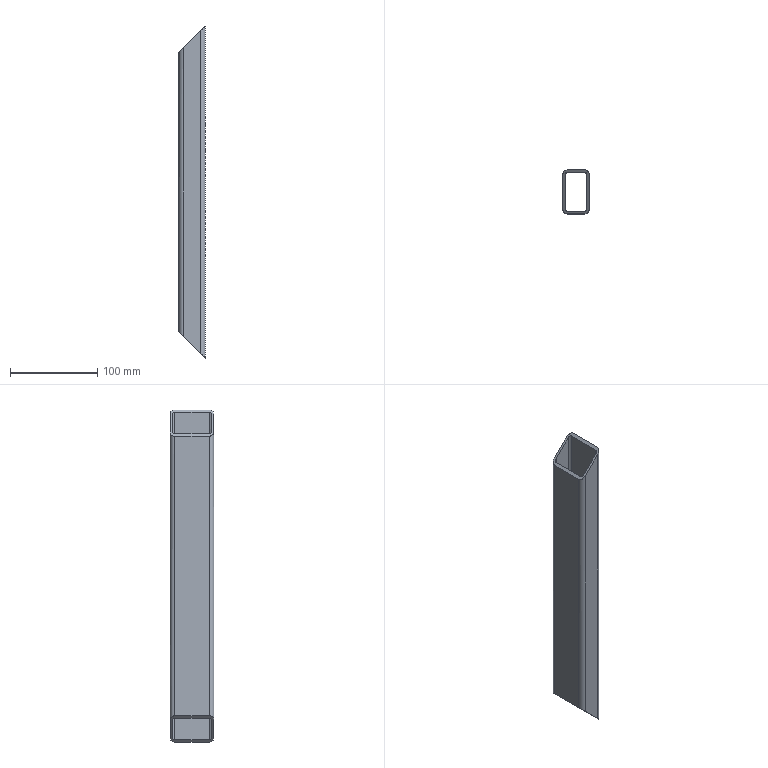Component | SolidWorks | Frame-1_SquareTube2-1 | 1 solid | 18 faces | box 30 x 50 x 380 mm | volume 130043 mm3 | plane 10 | cylinder 8 | commonest cylinder face diameters 10.4 x4 5.2 x4
STEP:
#1=COLOUR_RGB('',0.7922,0.8196,0.9333);
#2=FILL_AREA_STYLE_COLOUR('',#1);
#3=FILL_AREA_STYLE('',(#2));
#4=SURFACE_STYLE_FILL_AREA(#3);
#5=SURFACE_SIDE_STYLE('',(#4));
#6=SURFACE_STYLE_USAGE(.BOTH.,#5);
#7=PRESENTATION_STYLE_ASSIGNMENT((#6));
#8=CARTESIAN_POINT('',(20.276,-0.7795,-7.48));
#9=VERTEX_POINT('',#8);
#10=CARTESIAN_POINT('',(20.276,-0.7795,7.48));
#11=VERTEX_POINT('',#10);
#12=CARTESIAN_POINT('',(20.276,-0.7795,-6.89));
#13=DIRECTION('',(0.,0.,1.));
#14=VECTOR('',#13,39.37);
#15=LINE('',#12,#14);
#16=EDGE_CURVE('',#9,#11,#15,.T.);
#17=ORIENTED_EDGE('',*,*,#16,.F.);
#18=CARTESIAN_POINT('',(20.276,0.7795,-7.48));
#19=VERTEX_POINT('',#18);
#20=CARTESIAN_POINT('',(20.276,-0.7795,-7.48));
#21=DIRECTION('',(0.,-1.,0.));
#22=VECTOR('',#21,39.37);
#23=LINE('',#20,#22);
#24=EDGE_CURVE('',#19,#9,#23,.T.);
#25=ORIENTED_EDGE('',*,*,#24,.F.);
#26=CARTESIAN_POINT('',(20.276,0.7795,7.48));
#27=VERTEX_POINT('',#26);
#28=CARTESIAN_POINT('',(20.276,0.7795,-6.89));
#29=DIRECTION('',(0.,0.,-1.));
#30=VECTOR('',#29,39.37);
#31=LINE('',#28,#30);
#32=EDGE_CURVE('',#27,#19,#31,.T.);
#33=ORIENTED_EDGE('',*,*,#32,.F.);
#34=CARTESIAN_POINT('',(20.276,-0.7795,7.48));
#35=DIRECTION('',(0.,1.,0.));
#36=VECTOR('',#35,39.37);
#37=LINE('',#34,#36);
#38=EDGE_CURVE('',#11,#27,#37,.T.);
#39=ORIENTED_EDGE('',*,*,#38,.F.);
#40=EDGE_LOOP('',(#17,#25,#33,#39));
#41=FACE_OUTER_BOUND('',#40,.T.);
#42=CARTESIAN_POINT('',(20.276,-0.7795,-6.89));
#43=DIRECTION('',(-1.,0.,0.));
#44=DIRECTION('',(0.,0.,1.));
#45=AXIS2_PLACEMENT_3D('',#42,#43,#44);
#46=PLANE('',#45);
#47=ADVANCED_FACE('',(#41),#46,.F.);
#48=ORIENTED_EDGE('',*,*,#38,.T.);
#49=CARTESIAN_POINT('',(20.071,0.9843,7.276));
#50=VERTEX_POINT('',#49);
#51=CARTESIAN_POINT('',(20.276,0.7795,7.48));
#52=CARTESIAN_POINT('',(20.276,0.8995,7.48));
#53=CARTESIAN_POINT('',(20.191,0.9843,7.396));
#54=CARTESIAN_POINT('',(20.071,0.9843,7.276));
#55=(BOUNDED_CURVE()B_SPLINE_CURVE(3,(#51,#52,#53,#54),.UNSPECIFIED.,.F.,.F.)B_SPLINE_CURVE_WITH_KNOTS((4,4),(0.,1.571),.UNSPECIFIED.)CURVE()GEOMETRIC_REPRESENTATION_ITEM()RATIONAL_B_SPLINE_CURVE((1.,0.8047,0.8047,1.))REPRESENTATION_ITEM(''));
#56=EDGE_CURVE('',#27,#50,#55,.T.);
#57=ORIENTED_EDGE('',*,*,#56,.T.);
#58=CARTESIAN_POINT('',(19.299,0.9843,6.504));
#59=VERTEX_POINT('',#58);
#60=CARTESIAN_POINT('',(19.685,0.9843,6.89));
#61=DIRECTION('',(-0.7071,0.,-0.7071));
#62=VECTOR('',#61,39.37);
#63=LINE('',#60,#62);
#64=EDGE_CURVE('',#50,#59,#63,.T.);
#65=ORIENTED_EDGE('',*,*,#64,.T.);
#66=CARTESIAN_POINT('',(19.094,0.7795,6.299));
#67=VERTEX_POINT('',#66);
#68=CARTESIAN_POINT('',(19.299,0.9843,6.504));
#69=CARTESIAN_POINT('',(19.179,0.9843,6.384));
#70=CARTESIAN_POINT('',(19.094,0.8995,6.299));
#71=CARTESIAN_POINT('',(19.094,0.7795,6.299));
#72=(BOUNDED_CURVE()B_SPLINE_CURVE(3,(#68,#69,#70,#71),.UNSPECIFIED.,.F.,.T.)B_SPLINE_CURVE_WITH_KNOTS((4,4),(1.571,3.142),.UNSPECIFIED.)CURVE()GEOMETRIC_REPRESENTATION_ITEM()RATIONAL_B_SPLINE_CURVE((1.,0.8047,0.8047,1.))REPRESENTATION_ITEM(''));
#73=EDGE_CURVE('',#59,#67,#72,.T.);
#74=ORIENTED_EDGE('',*,*,#73,.T.);
#75=CARTESIAN_POINT('',(19.094,-0.7795,6.299));
#76=VERTEX_POINT('',#75);
#77=CARTESIAN_POINT('',(19.094,0.,6.299));
#78=DIRECTION('',(0.,-1.,0.));
#79=VECTOR('',#78,39.37);
#80=LINE('',#77,#79);
#81=EDGE_CURVE('',#67,#76,#80,.T.);
#82=ORIENTED_EDGE('',*,*,#81,.T.);
#83=CARTESIAN_POINT('',(19.299,-0.9843,6.504));
#84=VERTEX_POINT('',#83);
#85=CARTESIAN_POINT('',(19.094,-0.7795,6.299));
#86=CARTESIAN_POINT('',(19.094,-0.8995,6.299));
#87=CARTESIAN_POINT('',(19.179,-0.9843,6.384));
#88=CARTESIAN_POINT('',(19.299,-0.9843,6.504));
#89=(BOUNDED_CURVE()B_SPLINE_CURVE(3,(#85,#86,#87,#88),.UNSPECIFIED.,.F.,.F.)B_SPLINE_CURVE_WITH_KNOTS((4,4),(3.142,4.712),.UNSPECIFIED.)CURVE()GEOMETRIC_REPRESENTATION_ITEM()RATIONAL_B_SPLINE_CURVE((1.,0.8047,0.8047,1.))REPRESENTATION_ITEM(''));
#90=EDGE_CURVE('',#76,#84,#89,.T.);
#91=ORIENTED_EDGE('',*,*,#90,.T.);
#92=CARTESIAN_POINT('',(20.071,-0.9843,7.276));
#93=VERTEX_POINT('',#92);
#94=CARTESIAN_POINT('',(19.685,-0.9843,6.89));
#95=DIRECTION('',(0.7071,0.,0.7071));
#96=VECTOR('',#95,39.37);
#97=LINE('',#94,#96);
#98=EDGE_CURVE('',#84,#93,#97,.T.);
#99=ORIENTED_EDGE('',*,*,#98,.T.);
#100=CARTESIAN_POINT('',(20.071,-0.9843,7.276));
#101=CARTESIAN_POINT('',(20.191,-0.9843,7.396));
#102=CARTESIAN_POINT('',(20.276,-0.8995,7.48));
#103=CARTESIAN_POINT('',(20.276,-0.7795,7.48));
#104=(BOUNDED_CURVE()B_SPLINE_CURVE(3,(#100,#101,#102,#103),.UNSPECIFIED.,.F.,.F.)B_SPLINE_CURVE_WITH_KNOTS((4,4),(4.712,6.283),.UNSPECIFIED.)CURVE()GEOMETRIC_REPRESENTATION_ITEM()RATIONAL_B_SPLINE_CURVE((1.,0.8047,0.8047,1.))REPRESENTATION_ITEM(''));
#105=EDGE_CURVE('',#93,#11,#104,.T.);
#106=ORIENTED_EDGE('',*,*,#105,.T.);
#107=EDGE_LOOP('',(#48,#57,#65,#74,#82,#91,#99,#106));
#108=FACE_OUTER_BOUND('',#107,.T.);
#109=CARTESIAN_POINT('',(19.197,0.7795,6.402));
#110=VERTEX_POINT('',#109);
#111=CARTESIAN_POINT('',(19.299,0.8819,6.504));
#112=VERTEX_POINT('',#111);
#113=CARTESIAN_POINT('',(19.197,0.7795,6.402));
#114=CARTESIAN_POINT('',(19.197,0.8395,6.402));
#115=CARTESIAN_POINT('',(19.239,0.8819,6.444));
#116=CARTESIAN_POINT('',(19.299,0.8819,6.504));
#117=(BOUNDED_CURVE()B_SPLINE_CURVE(3,(#113,#114,#115,#116),.UNSPECIFIED.,.F.,.F.)B_SPLINE_CURVE_WITH_KNOTS((4,4),(3.142,4.712),.UNSPECIFIED.)CURVE()GEOMETRIC_REPRESENTATION_ITEM()RATIONAL_B_SPLINE_CURVE((1.,0.8047,0.8047,1.))REPRESENTATION_ITEM(''));
#118=EDGE_CURVE('',#110,#112,#117,.T.);
#119=ORIENTED_EDGE('',*,*,#118,.T.);
#120=CARTESIAN_POINT('',(20.071,0.8819,7.276));
#121=VERTEX_POINT('',#120);
#122=CARTESIAN_POINT('',(19.685,0.8819,6.89));
#123=DIRECTION('',(0.7071,0.,0.7071));
#124=VECTOR('',#123,39.37);
#125=LINE('',#122,#124);
#126=EDGE_CURVE('',#112,#121,#125,.T.);
#127=ORIENTED_EDGE('',*,*,#126,.T.);
#128=CARTESIAN_POINT('',(20.173,0.7795,7.378));
#129=VERTEX_POINT('',#128);
#130=CARTESIAN_POINT('',(20.071,0.8819,7.276));
#131=CARTESIAN_POINT('',(20.131,0.8819,7.336));
#132=CARTESIAN_POINT('',(20.173,0.8395,7.378));
#133=CARTESIAN_POINT('',(20.173,0.7795,7.378));
#134=(BOUNDED_CURVE()B_SPLINE_CURVE(3,(#130,#131,#132,#133),.UNSPECIFIED.,.F.,.F.)B_SPLINE_CURVE_WITH_KNOTS((4,4),(4.712,6.283),.UNSPECIFIED.)CURVE()GEOMETRIC_REPRESENTATION_ITEM()RATIONAL_B_SPLINE_CURVE((1.,0.8047,0.8047,1.))REPRESENTATION_ITEM(''));
#135=EDGE_CURVE('',#121,#129,#134,.T.);
#136=ORIENTED_EDGE('',*,*,#135,.T.);
#137=CARTESIAN_POINT('',(20.173,-0.7795,7.378));
#138=VERTEX_POINT('',#137);
#139=CARTESIAN_POINT('',(20.173,0.,7.378));
#140=DIRECTION('',(0.,-1.,0.));
#141=VECTOR('',#140,39.37);
#142=LINE('',#139,#141);
#143=EDGE_CURVE('',#129,#138,#142,.T.);
#144=ORIENTED_EDGE('',*,*,#143,.T.);
#145=CARTESIAN_POINT('',(20.071,-0.8819,7.276));
#146=VERTEX_POINT('',#145);
#147=CARTESIAN_POINT('',(20.173,-0.7795,7.378));
#148=CARTESIAN_POINT('',(20.173,-0.8395,7.378));
#149=CARTESIAN_POINT('',(20.131,-0.8819,7.336));
#150=CARTESIAN_POINT('',(20.071,-0.8819,7.276));
#151=(BOUNDED_CURVE()B_SPLINE_CURVE(3,(#147,#148,#149,#150),.UNSPECIFIED.,.F.,.F.)B_SPLINE_CURVE_WITH_KNOTS((4,4),(0.,1.571),.UNSPECIFIED.)CURVE()GEOMETRIC_REPRESENTATION_ITEM()RATIONAL_B_SPLINE_CURVE((1.,0.8047,0.8047,1.))REPRESENTATION_ITEM(''));
#152=EDGE_CURVE('',#138,#146,#151,.T.);
#153=ORIENTED_EDGE('',*,*,#152,.T.);
#154=CARTESIAN_POINT('',(19.299,-0.8819,6.504));
#155=VERTEX_POINT('',#154);
#156=CARTESIAN_POINT('',(19.685,-0.8819,6.89));
#157=DIRECTION('',(-0.7071,0.,-0.7071));
#158=VECTOR('',#157,39.37);
#159=LINE('',#156,#158);
#160=EDGE_CURVE('',#146,#155,#159,.T.);
#161=ORIENTED_EDGE('',*,*,#160,.T.);
#162=CARTESIAN_POINT('',(19.197,-0.7795,6.402));
#163=VERTEX_POINT('',#162);
#164=CARTESIAN_POINT('',(19.299,-0.8819,6.504));
#165=CARTESIAN_POINT('',(19.239,-0.8819,6.444));
#166=CARTESIAN_POINT('',(19.197,-0.8395,6.402));
#167=CARTESIAN_POINT('',(19.197,-0.7795,6.402));
#168=(BOUNDED_CURVE()B_SPLINE_CURVE(3,(#164,#165,#166,#167),.UNSPECIFIED.,.F.,.F.)B_SPLINE_CURVE_WITH_KNOTS((4,4),(1.571,3.142),.UNSPECIFIED.)CURVE()GEOMETRIC_REPRESENTATION_ITEM()RATIONAL_B_SPLINE_CURVE((1.,0.8047,0.8047,1.))REPRESENTATION_ITEM(''));
#169=EDGE_CURVE('',#155,#163,#168,.T.);
#170=ORIENTED_EDGE('',*,*,#169,.T.);
#171=CARTESIAN_POINT('',(19.197,0.,6.402));
#172=DIRECTION('',(0.,1.,0.));
#173=VECTOR('',#172,39.37);
#174=LINE('',#171,#173);
#175=EDGE_CURVE('',#163,#110,#174,.T.);
#176=ORIENTED_EDGE('',*,*,#175,.T.);
#177=EDGE_LOOP('',(#119,#127,#136,#144,#153,#161,#170,#176));
#178=FACE_BOUND('',#177,.T.);
#179=CARTESIAN_POINT('',(19.685,0.,6.89));
#180=DIRECTION('',(-0.7071,0.,0.7071));
#181=DIRECTION('',(0.7071,0.,0.7071));
#182=AXIS2_PLACEMENT_3D('',#179,#180,#181);
#183=PLANE('',#182);
#184=ADVANCED_FACE('',(#108,#178),#183,.T.);
#185=CARTESIAN_POINT('',(20.071,-0.9843,-7.276));
#186=VERTEX_POINT('',#185);
#187=CARTESIAN_POINT('',(20.071,-0.9843,-7.276));
#188=CARTESIAN_POINT('',(20.191,-0.9843,-7.396));
#189=CARTESIAN_POINT('',(20.276,-0.8995,-7.48));
#190=CARTESIAN_POINT('',(20.276,-0.7795,-7.48));
#191=(BOUNDED_CURVE()B_SPLINE_CURVE(3,(#187,#188,#189,#190),.UNSPECIFIED.,.F.,.F.)B_SPLINE_CURVE_WITH_KNOTS((4,4),(1.571,3.142),.UNSPECIFIED.)CURVE()GEOMETRIC_REPRESENTATION_ITEM()RATIONAL_B_SPLINE_CURVE((1.,0.8047,0.8047,1.))REPRESENTATION_ITEM(''));
#192=EDGE_CURVE('',#186,#9,#191,.T.);
#193=ORIENTED_EDGE('',*,*,#192,.T.);
#194=ORIENTED_EDGE('',*,*,#16,.T.);
#195=ORIENTED_EDGE('',*,*,#105,.F.);
#196=CARTESIAN_POINT('',(20.071,-0.9843,-6.89));
#197=DIRECTION('',(0.,0.,-1.));
#198=VECTOR('',#197,39.37);
#199=LINE('',#196,#198);
#200=EDGE_CURVE('',#93,#186,#199,.T.);
#201=ORIENTED_EDGE('',*,*,#200,.T.);
#202=EDGE_LOOP('',(#193,#194,#195,#201));
#203=FACE_OUTER_BOUND('',#202,.T.);
#204=CARTESIAN_POINT('',(20.071,-0.7795,-6.89));
#205=DIRECTION('',(0.,0.,1.));
#206=DIRECTION('',(1.,0.,0.));
#207=AXIS2_PLACEMENT_3D('',#204,#205,#206);
#208=CYLINDRICAL_SURFACE('',#207,0.2047);
#209=ADVANCED_FACE('',(#203),#208,.T.);
#210=CARTESIAN_POINT('',(19.299,-0.9843,-6.504));
#211=VERTEX_POINT('',#210);
#212=CARTESIAN_POINT('',(19.685,-0.9843,-6.89));
#213=DIRECTION('',(-0.7071,0.,0.7071));
#214=VECTOR('',#213,39.37);
#215=LINE('',#212,#214);
#216=EDGE_CURVE('',#186,#211,#215,.T.);
#217=ORIENTED_EDGE('',*,*,#216,.T.);
#218=CARTESIAN_POINT('',(19.094,-0.7795,-6.299));
#219=VERTEX_POINT('',#218);
#220=CARTESIAN_POINT('',(19.299,-0.9843,-6.504));
#221=CARTESIAN_POINT('',(19.179,-0.9843,-6.384));
#222=CARTESIAN_POINT('',(19.094,-0.8995,-6.299));
#223=CARTESIAN_POINT('',(19.094,-0.7795,-6.299));
#224=(BOUNDED_CURVE()B_SPLINE_CURVE(3,(#220,#221,#222,#223),.UNSPECIFIED.,.F.,.F.)B_SPLINE_CURVE_WITH_KNOTS((4,4),(4.712,6.283),.UNSPECIFIED.)CURVE()GEOMETRIC_REPRESENTATION_ITEM()RATIONAL_B_SPLINE_CURVE((1.,0.8047,0.8047,1.))REPRESENTATION_ITEM(''));
#225=EDGE_CURVE('',#211,#219,#224,.T.);
#226=ORIENTED_EDGE('',*,*,#225,.T.);
#227=CARTESIAN_POINT('',(19.094,0.7795,-6.299));
#228=VERTEX_POINT('',#227);
#229=CARTESIAN_POINT('',(19.094,0.,-6.299));
#230=DIRECTION('',(0.,1.,0.));
#231=VECTOR('',#230,39.37);
#232=LINE('',#229,#231);
#233=EDGE_CURVE('',#219,#228,#232,.T.);
#234=ORIENTED_EDGE('',*,*,#233,.T.);
#235=CARTESIAN_POINT('',(19.299,0.9843,-6.504));
#236=VERTEX_POINT('',#235);
#237=CARTESIAN_POINT('',(19.094,0.7795,-6.299));
#238=CARTESIAN_POINT('',(19.094,0.8995,-6.299));
#239=CARTESIAN_POINT('',(19.179,0.9843,-6.384));
#240=CARTESIAN_POINT('',(19.299,0.9843,-6.504));
#241=(BOUNDED_CURVE()B_SPLINE_CURVE(3,(#237,#238,#239,#240),.UNSPECIFIED.,.F.,.F.)B_SPLINE_CURVE_WITH_KNOTS((4,4),(0.,1.571),.UNSPECIFIED.)CURVE()GEOMETRIC_REPRESENTATION_ITEM()RATIONAL_B_SPLINE_CURVE((1.,0.8047,0.8047,1.))REPRESENTATION_ITEM(''));
#242=EDGE_CURVE('',#228,#236,#241,.T.);
#243=ORIENTED_EDGE('',*,*,#242,.T.);
#244=CARTESIAN_POINT('',(20.071,0.9843,-7.276));
#245=VERTEX_POINT('',#244);
#246=CARTESIAN_POINT('',(19.685,0.9843,-6.89));
#247=DIRECTION('',(0.7071,0.,-0.7071));
#248=VECTOR('',#247,39.37);
#249=LINE('',#246,#248);
#250=EDGE_CURVE('',#236,#245,#249,.T.);
#251=ORIENTED_EDGE('',*,*,#250,.T.);
#252=CARTESIAN_POINT('',(20.071,0.9843,-7.276));
#253=CARTESIAN_POINT('',(20.191,0.9843,-7.396));
#254=CARTESIAN_POINT('',(20.276,0.8995,-7.48));
#255=CARTESIAN_POINT('',(20.276,0.7795,-7.48));
#256=(BOUNDED_CURVE()B_SPLINE_CURVE(3,(#252,#253,#254,#255),.UNSPECIFIED.,.F.,.T.)B_SPLINE_CURVE_WITH_KNOTS((4,4),(1.571,3.142),.UNSPECIFIED.)CURVE()GEOMETRIC_REPRESENTATION_ITEM()RATIONAL_B_SPLINE_CURVE((1.,0.8047,0.8047,1.))REPRESENTATION_ITEM(''));
#257=EDGE_CURVE('',#245,#19,#256,.T.);
#258=ORIENTED_EDGE('',*,*,#257,.T.);
#259=ORIENTED_EDGE('',*,*,#24,.T.);
#260=ORIENTED_EDGE('',*,*,#192,.F.);
#261=EDGE_LOOP('',(#217,#226,#234,#243,#251,#258,#259,#260));
#262=FACE_OUTER_BOUND('',#261,.T.);
#263=CARTESIAN_POINT('',(20.071,-0.8819,-7.276));
#264=VERTEX_POINT('',#263);
#265=CARTESIAN_POINT('',(20.173,-0.7795,-7.378));
#266=VERTEX_POINT('',#265);
#267=CARTESIAN_POINT('',(20.071,-0.8819,-7.276));
#268=CARTESIAN_POINT('',(20.131,-0.8819,-7.336));
#269=CARTESIAN_POINT('',(20.173,-0.8395,-7.378));
#270=CARTESIAN_POINT('',(20.173,-0.7795,-7.378));
#271=(BOUNDED_CURVE()B_SPLINE_CURVE(3,(#267,#268,#269,#270),.UNSPECIFIED.,.F.,.F.)B_SPLINE_CURVE_WITH_KNOTS((4,4),(1.571,3.142),.UNSPECIFIED.)CURVE()GEOMETRIC_REPRESENTATION_ITEM()RATIONAL_B_SPLINE_CURVE((1.,0.8047,0.8047,1.))REPRESENTATION_ITEM(''));
#272=EDGE_CURVE('',#264,#266,#271,.T.);
#273=ORIENTED_EDGE('',*,*,#272,.T.);
#274=CARTESIAN_POINT('',(20.173,0.7795,-7.378));
#275=VERTEX_POINT('',#274);
#276=CARTESIAN_POINT('',(20.173,0.,-7.378));
#277=DIRECTION('',(0.,1.,0.));
#278=VECTOR('',#277,39.37);
#279=LINE('',#276,#278);
#280=EDGE_CURVE('',#266,#275,#279,.T.);
#281=ORIENTED_EDGE('',*,*,#280,.T.);
#282=CARTESIAN_POINT('',(20.071,0.8819,-7.276));
#283=VERTEX_POINT('',#282);
#284=CARTESIAN_POINT('',(20.173,0.7795,-7.378));
#285=CARTESIAN_POINT('',(20.173,0.8395,-7.378));
#286=CARTESIAN_POINT('',(20.131,0.8819,-7.336));
#287=CARTESIAN_POINT('',(20.071,0.8819,-7.276));
#288=(BOUNDED_CURVE()B_SPLINE_CURVE(3,(#284,#285,#286,#287),.UNSPECIFIED.,.F.,.F.)B_SPLINE_CURVE_WITH_KNOTS((4,4),(3.142,4.712),.UNSPECIFIED.)CURVE()GEOMETRIC_REPRESENTATION_ITEM()RATIONAL_B_SPLINE_CURVE((1.,0.8047,0.8047,1.))REPRESENTATION_ITEM(''));
#289=EDGE_CURVE('',#275,#283,#288,.T.);
#290=ORIENTED_EDGE('',*,*,#289,.T.);
#291=CARTESIAN_POINT('',(19.299,0.8819,-6.504));
#292=VERTEX_POINT('',#291);
#293=CARTESIAN_POINT('',(19.685,0.8819,-6.89));
#294=DIRECTION('',(-0.7071,0.,0.7071));
#295=VECTOR('',#294,39.37);
#296=LINE('',#293,#295);
#297=EDGE_CURVE('',#283,#292,#296,.T.);
#298=ORIENTED_EDGE('',*,*,#297,.T.);
#299=CARTESIAN_POINT('',(19.197,0.7795,-6.402));
#300=VERTEX_POINT('',#299);
#301=CARTESIAN_POINT('',(19.299,0.8819,-6.504));
#302=CARTESIAN_POINT('',(19.239,0.8819,-6.444));
#303=CARTESIAN_POINT('',(19.197,0.8395,-6.402));
#304=CARTESIAN_POINT('',(19.197,0.7795,-6.402));
#305=(BOUNDED_CURVE()B_SPLINE_CURVE(3,(#301,#302,#303,#304),.UNSPECIFIED.,.F.,.F.)B_SPLINE_CURVE_WITH_KNOTS((4,4),(4.712,6.283),.UNSPECIFIED.)CURVE()GEOMETRIC_REPRESENTATION_ITEM()RATIONAL_B_SPLINE_CURVE((1.,0.8047,0.8047,1.))REPRESENTATION_ITEM(''));
#306=EDGE_CURVE('',#292,#300,#305,.T.);
#307=ORIENTED_EDGE('',*,*,#306,.T.);
#308=CARTESIAN_POINT('',(19.197,-0.7795,-6.402));
#309=VERTEX_POINT('',#308);
#310=CARTESIAN_POINT('',(19.197,0.,-6.402));
#311=DIRECTION('',(0.,-1.,0.));
#312=VECTOR('',#311,39.37);
#313=LINE('',#310,#312);
#314=EDGE_CURVE('',#300,#309,#313,.T.);
#315=ORIENTED_EDGE('',*,*,#314,.T.);
#316=CARTESIAN_POINT('',(19.299,-0.8819,-6.504));
#317=VERTEX_POINT('',#316);
#318=CARTESIAN_POINT('',(19.197,-0.7795,-6.402));
#319=CARTESIAN_POINT('',(19.197,-0.8395,-6.402));
#320=CARTESIAN_POINT('',(19.239,-0.8819,-6.444));
#321=CARTESIAN_POINT('',(19.299,-0.8819,-6.504));
#322=(BOUNDED_CURVE()B_SPLINE_CURVE(3,(#318,#319,#320,#321),.UNSPECIFIED.,.F.,.F.)B_SPLINE_CURVE_WITH_KNOTS((4,4),(0.,1.571),.UNSPECIFIED.)CURVE()GEOMETRIC_REPRESENTATION_ITEM()RATIONAL_B_SPLINE_CURVE((1.,0.8047,0.8047,1.))REPRESENTATION_ITEM(''));
#323=EDGE_CURVE('',#309,#317,#322,.T.);
#324=ORIENTED_EDGE('',*,*,#323,.T.);
#325=CARTESIAN_POINT('',(19.685,-0.8819,-6.89));
#326=DIRECTION('',(0.7071,0.,-0.7071));
#327=VECTOR('',#326,39.37);
#328=LINE('',#325,#327);
#329=EDGE_CURVE('',#317,#264,#328,.T.);
#330=ORIENTED_EDGE('',*,*,#329,.T.);
#331=EDGE_LOOP('',(#273,#281,#290,#298,#307,#315,#324,#330));
#332=FACE_BOUND('',#331,.T.);
#333=CARTESIAN_POINT('',(19.685,0.,-6.89));
#334=DIRECTION('',(-0.7071,0.,-0.7071));
#335=DIRECTION('',(-0.7071,0.,0.7071));
#336=AXIS2_PLACEMENT_3D('',#333,#334,#335);
#337=PLANE('',#336);
#338=ADVANCED_FACE('',(#262,#332),#337,.T.);
#339=ORIENTED_EDGE('',*,*,#257,.F.);
#340=CARTESIAN_POINT('',(20.071,0.9843,-6.89));
#341=DIRECTION('',(0.,0.,1.));
#342=VECTOR('',#341,39.37);
#343=LINE('',#340,#342);
#344=EDGE_CURVE('',#245,#50,#343,.T.);
#345=ORIENTED_EDGE('',*,*,#344,.T.);
#346=ORIENTED_EDGE('',*,*,#56,.F.);
#347=ORIENTED_EDGE('',*,*,#32,.T.);
#348=EDGE_LOOP('',(#339,#345,#346,#347));
#349=FACE_OUTER_BOUND('',#348,.T.);
#350=CARTESIAN_POINT('',(20.071,0.7795,-6.89));
#351=DIRECTION('',(0.,0.,1.));
#352=DIRECTION('',(1.,0.,0.));
#353=AXIS2_PLACEMENT_3D('',#350,#351,#352);
#354=CYLINDRICAL_SURFACE('',#353,0.2047);
#355=ADVANCED_FACE('',(#349),#354,.T.);
#356=CARTESIAN_POINT('',(19.299,-0.9843,-6.89));
#357=DIRECTION('',(0.,0.,1.));
#358=VECTOR('',#357,39.37);
#359=LINE('',#356,#358);
#360=EDGE_CURVE('',#211,#84,#359,.T.);
#361=ORIENTED_EDGE('',*,*,#360,.F.);
#362=ORIENTED_EDGE('',*,*,#216,.F.);
#363=ORIENTED_EDGE('',*,*,#200,.F.);
#364=ORIENTED_EDGE('',*,*,#98,.F.);
#365=EDGE_LOOP('',(#361,#362,#363,#364));
#366=FACE_OUTER_BOUND('',#365,.T.);
#367=CARTESIAN_POINT('',(20.071,-0.9843,-6.89));
#368=DIRECTION('',(0.,1.,0.));
#369=DIRECTION('',(0.,0.,1.));
#370=AXIS2_PLACEMENT_3D('',#367,#368,#369);
#371=PLANE('',#370);
#372=ADVANCED_FACE('',(#366),#371,.F.);
#373=ORIENTED_EDGE('',*,*,#225,.F.);
#374=ORIENTED_EDGE('',*,*,#360,.T.);
#375=ORIENTED_EDGE('',*,*,#90,.F.);
#376=CARTESIAN_POINT('',(19.094,-0.7795,-6.89));
#377=DIRECTION('',(0.,0.,-1.));
#378=VECTOR('',#377,39.37);
#379=LINE('',#376,#378);
#380=EDGE_CURVE('',#76,#219,#379,.T.);
#381=ORIENTED_EDGE('',*,*,#380,.T.);
#382=EDGE_LOOP('',(#373,#374,#375,#381));
#383=FACE_OUTER_BOUND('',#382,.T.);
#384=CARTESIAN_POINT('',(19.299,-0.7795,-6.89));
#385=DIRECTION('',(0.,0.,1.));
#386=DIRECTION('',(1.,0.,0.));
#387=AXIS2_PLACEMENT_3D('',#384,#385,#386);
#388=CYLINDRICAL_SURFACE('',#387,0.2047);
#389=ADVANCED_FACE('',(#383),#388,.T.);
#390=CARTESIAN_POINT('',(19.094,0.7795,-6.89));
#391=DIRECTION('',(0.,0.,1.));
#392=VECTOR('',#391,39.37);
#393=LINE('',#390,#392);
#394=EDGE_CURVE('',#228,#67,#393,.T.);
#395=ORIENTED_EDGE('',*,*,#394,.F.);
#396=ORIENTED_EDGE('',*,*,#233,.F.);
#397=ORIENTED_EDGE('',*,*,#380,.F.);
#398=ORIENTED_EDGE('',*,*,#81,.F.);
#399=EDGE_LOOP('',(#395,#396,#397,#398));
#400=FACE_OUTER_BOUND('',#399,.T.);
#401=CARTESIAN_POINT('',(19.094,0.7795,-6.89));
#402=DIRECTION('',(1.,0.,0.));
#403=DIRECTION('',(0.,0.,-1.));
#404=AXIS2_PLACEMENT_3D('',#401,#402,#403);
#405=PLANE('',#404);
#406=ADVANCED_FACE('',(#400),#405,.F.);
#407=ORIENTED_EDGE('',*,*,#242,.F.);
#408=ORIENTED_EDGE('',*,*,#394,.T.);
#409=ORIENTED_EDGE('',*,*,#73,.F.);
#410=CARTESIAN_POINT('',(19.299,0.9843,-6.89));
#411=DIRECTION('',(0.,0.,-1.));
#412=VECTOR('',#411,39.37);
#413=LINE('',#410,#412);
#414=EDGE_CURVE('',#59,#236,#413,.T.);
#415=ORIENTED_EDGE('',*,*,#414,.T.);
#416=EDGE_LOOP('',(#407,#408,#409,#415));
#417=FACE_OUTER_BOUND('',#416,.T.);
#418=CARTESIAN_POINT('',(19.299,0.7795,-6.89));
#419=DIRECTION('',(0.,0.,1.));
#420=DIRECTION('',(1.,0.,0.));
#421=AXIS2_PLACEMENT_3D('',#418,#419,#420);
#422=CYLINDRICAL_SURFACE('',#421,0.2047);
#423=ADVANCED_FACE('',(#417),#422,.T.);
#424=ORIENTED_EDGE('',*,*,#344,.F.);
#425=ORIENTED_EDGE('',*,*,#250,.F.);
#426=ORIENTED_EDGE('',*,*,#414,.F.);
#427=ORIENTED_EDGE('',*,*,#64,.F.);
#428=EDGE_LOOP('',(#424,#425,#426,#427));
#429=FACE_OUTER_BOUND('',#428,.T.);
#430=CARTESIAN_POINT('',(19.299,0.9843,-6.89));
#431=DIRECTION('',(0.,-1.,0.));
#432=DIRECTION('',(0.,0.,-1.));
#433=AXIS2_PLACEMENT_3D('',#430,#431,#432);
#434=PLANE('',#433);
#435=ADVANCED_FACE('',(#429),#434,.F.);
#436=CARTESIAN_POINT('',(19.299,0.8819,-6.89));
#437=DIRECTION('',(0.,0.,-1.));
#438=VECTOR('',#437,39.37);
#439=LINE('',#436,#438);
#440=EDGE_CURVE('',#112,#292,#439,.T.);
#441=ORIENTED_EDGE('',*,*,#440,.T.);
#442=ORIENTED_EDGE('',*,*,#297,.F.);
#443=CARTESIAN_POINT('',(20.071,0.8819,-6.89));
#444=DIRECTION('',(0.,0.,1.));
#445=VECTOR('',#444,39.37);
#446=LINE('',#443,#445);
#447=EDGE_CURVE('',#283,#121,#446,.T.);
#448=ORIENTED_EDGE('',*,*,#447,.T.);
#449=ORIENTED_EDGE('',*,*,#126,.F.);
#450=EDGE_LOOP('',(#441,#442,#448,#449));
#451=FACE_OUTER_BOUND('',#450,.T.);
#452=CARTESIAN_POINT('',(19.299,0.8819,-6.89));
#453=DIRECTION('',(0.,-1.,0.));
#454=DIRECTION('',(0.,0.,-1.));
#455=AXIS2_PLACEMENT_3D('',#452,#453,#454);
#456=PLANE('',#455);
#457=ADVANCED_FACE('',(#451),#456,.T.);
#458=ORIENTED_EDGE('',*,*,#118,.F.);
#459=CARTESIAN_POINT('',(19.197,0.7795,-6.89));
#460=DIRECTION('',(0.,0.,1.));
#461=VECTOR('',#460,39.37);
#462=LINE('',#459,#461);
#463=EDGE_CURVE('',#300,#110,#462,.T.);
#464=ORIENTED_EDGE('',*,*,#463,.F.);
#465=ORIENTED_EDGE('',*,*,#306,.F.);
#466=ORIENTED_EDGE('',*,*,#440,.F.);
#467=EDGE_LOOP('',(#458,#464,#465,#466));
#468=FACE_OUTER_BOUND('',#467,.T.);
#469=CARTESIAN_POINT('',(19.299,0.7795,-6.89));
#470=DIRECTION('',(0.,0.,1.));
#471=DIRECTION('',(1.,0.,0.));
#472=AXIS2_PLACEMENT_3D('',#469,#470,#471);
#473=CYLINDRICAL_SURFACE('',#472,0.1024);
#474=ADVANCED_FACE('',(#468),#473,.F.);
#475=CARTESIAN_POINT('',(19.197,-0.7795,-6.89));
#476=DIRECTION('',(0.,0.,-1.));
#477=VECTOR('',#476,39.37);
#478=LINE('',#475,#477);
#479=EDGE_CURVE('',#163,#309,#478,.T.);
#480=ORIENTED_EDGE('',*,*,#479,.T.);
#481=ORIENTED_EDGE('',*,*,#314,.F.);
#482=ORIENTED_EDGE('',*,*,#463,.T.);
#483=ORIENTED_EDGE('',*,*,#175,.F.);
#484=EDGE_LOOP('',(#480,#481,#482,#483));
#485=FACE_OUTER_BOUND('',#484,.T.);
#486=CARTESIAN_POINT('',(19.197,0.7795,-6.89));
#487=DIRECTION('',(1.,0.,0.));
#488=DIRECTION('',(0.,0.,-1.));
#489=AXIS2_PLACEMENT_3D('',#486,#487,#488);
#490=PLANE('',#489);
#491=ADVANCED_FACE('',(#485),#490,.T.);
#492=ORIENTED_EDGE('',*,*,#169,.F.);
#493=CARTESIAN_POINT('',(19.299,-0.8819,-6.89));
#494=DIRECTION('',(0.,0.,1.));
#495=VECTOR('',#494,39.37);
#496=LINE('',#493,#495);
#497=EDGE_CURVE('',#317,#155,#496,.T.);
#498=ORIENTED_EDGE('',*,*,#497,.F.);
#499=ORIENTED_EDGE('',*,*,#323,.F.);
#500=ORIENTED_EDGE('',*,*,#479,.F.);
#501=EDGE_LOOP('',(#492,#498,#499,#500));
#502=FACE_OUTER_BOUND('',#501,.T.);
#503=CARTESIAN_POINT('',(19.299,-0.7795,-6.89));
#504=DIRECTION('',(0.,0.,1.));
#505=DIRECTION('',(1.,0.,0.));
#506=AXIS2_PLACEMENT_3D('',#503,#504,#505);
#507=CYLINDRICAL_SURFACE('',#506,0.1024);
#508=ADVANCED_FACE('',(#502),#507,.F.);
#509=CARTESIAN_POINT('',(20.071,-0.8819,-6.89));
#510=DIRECTION('',(0.,0.,-1.));
#511=VECTOR('',#510,39.37);
#512=LINE('',#509,#511);
#513=EDGE_CURVE('',#146,#264,#512,.T.);
#514=ORIENTED_EDGE('',*,*,#513,.T.);
#515=ORIENTED_EDGE('',*,*,#329,.F.);
#516=ORIENTED_EDGE('',*,*,#497,.T.);
#517=ORIENTED_EDGE('',*,*,#160,.F.);
#518=EDGE_LOOP('',(#514,#515,#516,#517));
#519=FACE_OUTER_BOUND('',#518,.T.);
#520=CARTESIAN_POINT('',(20.071,-0.8819,-6.89));
#521=DIRECTION('',(0.,1.,0.));
#522=DIRECTION('',(0.,0.,1.));
#523=AXIS2_PLACEMENT_3D('',#520,#521,#522);
#524=PLANE('',#523);
#525=ADVANCED_FACE('',(#519),#524,.T.);
#526=ORIENTED_EDGE('',*,*,#152,.F.);
#527=CARTESIAN_POINT('',(20.173,-0.7795,-6.89));
#528=DIRECTION('',(0.,0.,1.));
#529=VECTOR('',#528,39.37);
#530=LINE('',#527,#529);
#531=EDGE_CURVE('',#266,#138,#530,.T.);
#532=ORIENTED_EDGE('',*,*,#531,.F.);
#533=ORIENTED_EDGE('',*,*,#272,.F.);
#534=ORIENTED_EDGE('',*,*,#513,.F.);
#535=EDGE_LOOP('',(#526,#532,#533,#534));
#536=FACE_OUTER_BOUND('',#535,.T.);
#537=CARTESIAN_POINT('',(20.071,-0.7795,-6.89));
#538=DIRECTION('',(0.,0.,1.));
#539=DIRECTION('',(1.,0.,0.));
#540=AXIS2_PLACEMENT_3D('',#537,#538,#539);
#541=CYLINDRICAL_SURFACE('',#540,0.1024);
#542=ADVANCED_FACE('',(#536),#541,.F.);
#543=CARTESIAN_POINT('',(20.173,0.7795,-6.89));
#544=DIRECTION('',(0.,0.,-1.));
#545=VECTOR('',#544,39.37);
#546=LINE('',#543,#545);
#547=EDGE_CURVE('',#129,#275,#546,.T.);
#548=ORIENTED_EDGE('',*,*,#547,.T.);
#549=ORIENTED_EDGE('',*,*,#280,.F.);
#550=ORIENTED_EDGE('',*,*,#531,.T.);
#551=ORIENTED_EDGE('',*,*,#143,.F.);
#552=EDGE_LOOP('',(#548,#549,#550,#551));
#553=FACE_OUTER_BOUND('',#552,.T.);
#554=CARTESIAN_POINT('',(20.173,-0.7795,-6.89));
#555=DIRECTION('',(-1.,0.,0.));
#556=DIRECTION('',(0.,0.,1.));
#557=AXIS2_PLACEMENT_3D('',#554,#555,#556);
#558=PLANE('',#557);
#559=ADVANCED_FACE('',(#553),#558,.T.);
#560=ORIENTED_EDGE('',*,*,#135,.F.);
#561=ORIENTED_EDGE('',*,*,#447,.F.);
#562=ORIENTED_EDGE('',*,*,#289,.F.);
#563=ORIENTED_EDGE('',*,*,#547,.F.);
#564=EDGE_LOOP('',(#560,#561,#562,#563));
#565=FACE_OUTER_BOUND('',#564,.T.);
#566=CARTESIAN_POINT('',(20.071,0.7795,-6.89));
#567=DIRECTION('',(0.,0.,1.));
#568=DIRECTION('',(1.,0.,0.));
#569=AXIS2_PLACEMENT_3D('',#566,#567,#568);
#570=CYLINDRICAL_SURFACE('',#569,0.1024);
#571=ADVANCED_FACE('',(#565),#570,.F.);
#572=CLOSED_SHELL('',(#47,#184,#209,#338,#355,#372,#389,#406,#423,#435,#457,#474,#491,#508,#525,#542,#559,#571));
#573=MANIFOLD_SOLID_BREP('',#572);
#574=STYLED_ITEM('',(#7),#573);
#575=(LENGTH_UNIT()NAMED_UNIT(*)SI_UNIT($,.METRE.));
#576=LENGTH_MEASURE_WITH_UNIT(LENGTH_MEASURE(0.0254),#575);
#577=DIMENSIONAL_EXPONENTS(1.,0.,0.,0.,0.,0.,0.);
#578=(CONVERSION_BASED_UNIT('',#576)LENGTH_UNIT()NAMED_UNIT(#577));
#579=UNCERTAINTY_MEASURE_WITH_UNIT(LENGTH_MEASURE(0.00001),#578,'','');
#580=(NAMED_UNIT(*)PLANE_ANGLE_UNIT()SI_UNIT($,.RADIAN.));
#581=(NAMED_UNIT(*)SI_UNIT($,.STERADIAN.)SOLID_ANGLE_UNIT());
#582=(GEOMETRIC_REPRESENTATION_CONTEXT(3)GLOBAL_UNCERTAINTY_ASSIGNED_CONTEXT((#579))GLOBAL_UNIT_ASSIGNED_CONTEXT((#578,#580,#581))REPRESENTATION_CONTEXT('',''));
#583=MECHANICAL_DESIGN_GEOMETRIC_PRESENTATION_REPRESENTATION('',(#574),#582);
#584=PRESENTATION_LAYER_ASSIGNMENT('','',(#574));
#585=CARTESIAN_POINT('',(0.,0.,0.));
#586=DIRECTION('',(0.,0.,1.));
#587=DIRECTION('',(1.,0.,0.));
#588=AXIS2_PLACEMENT_3D('',#585,#586,#587);
#589=(LENGTH_UNIT()NAMED_UNIT(*)SI_UNIT($,.METRE.));
#590=LENGTH_MEASURE_WITH_UNIT(LENGTH_MEASURE(0.0254),#589);
#591=DIMENSIONAL_EXPONENTS(1.,0.,0.,0.,0.,0.,0.);
#592=(CONVERSION_BASED_UNIT('',#590)LENGTH_UNIT()NAMED_UNIT(#591));
#593=UNCERTAINTY_MEASURE_WITH_UNIT(LENGTH_MEASURE(0.00001),#592,'','');
#594=(NAMED_UNIT(*)PLANE_ANGLE_UNIT()SI_UNIT($,.RADIAN.));
#595=(NAMED_UNIT(*)SI_UNIT($,.STERADIAN.)SOLID_ANGLE_UNIT());
#596=(GEOMETRIC_REPRESENTATION_CONTEXT(3)GLOBAL_UNCERTAINTY_ASSIGNED_CONTEXT((#593))GLOBAL_UNIT_ASSIGNED_CONTEXT((#592,#594,#595))REPRESENTATION_CONTEXT('',''));
#597=ADVANCED_BREP_SHAPE_REPRESENTATION('',(#573,#588),#596);